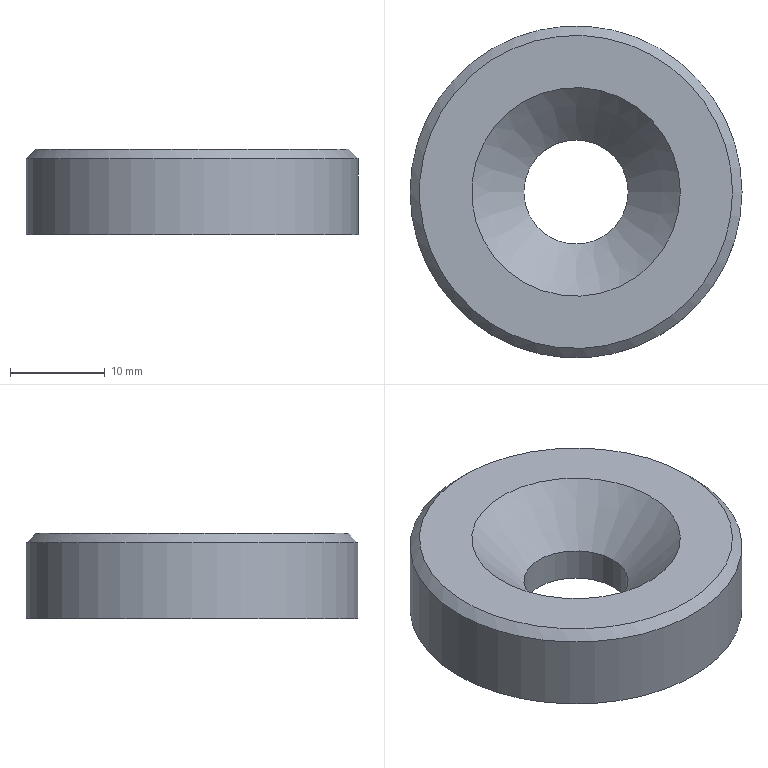Component | NX | END_CAP | 1 solid | 6 faces | box 35 x 35 x 9 mm | volume 7053 mm3 | plane 2 | cylinder 2 | cone 2 | commonest cylinder face diameters 35 x1 11 x1
STEP:
#1=CARTESIAN_POINT('',(0.,0.,0.));
#2=DIRECTION('',(0.,0.,1.));
#3=DIRECTION('',(1.,0.,0.));
#4=AXIS2_PLACEMENT_3D('',#1,#2,#3);
#5=CARTESIAN_POINT('',(16.5,0.,237.));
#6=VERTEX_POINT('',#5);
#7=CARTESIAN_POINT('',(-0.,0.,237.));
#8=DIRECTION('',(0.,0.,1.));
#9=DIRECTION('',(1.,0.,0.));
#10=AXIS2_PLACEMENT_3D('',#7,#8,#9);
#11=CIRCLE('',#10,16.5);
#12=CARTESIAN_POINT('',(-0.,0.,237.));
#13=DIRECTION('',(0.,0.,1.));
#14=DIRECTION('',(1.,0.,0.));
#15=AXIS2_PLACEMENT_3D('',#12,#13,#14);
#16=PLANE('',#15);
#17=CARTESIAN_POINT('',(0.,0.));
#18=DIRECTION('',(1.,0.));
#19=AXIS2_PLACEMENT_2D('',#17,#18);
#20=CIRCLE('',#19,16.5);
#21=(GEOMETRIC_REPRESENTATION_CONTEXT(2)PARAMETRIC_REPRESENTATION_CONTEXT()REPRESENTATION_CONTEXT('',''));
#22=DEFINITIONAL_REPRESENTATION('',(#20),#21);
#23=PCURVE('',#16,#22);
#24=CARTESIAN_POINT('',(-0.,0.,236.));
#25=DIRECTION('',(0.,0.,-1.));
#26=DIRECTION('',(-1.,0.,0.));
#27=AXIS2_PLACEMENT_3D('',#24,#25,#26);
#28=CONICAL_SURFACE('',#27,17.5,0.7854);
#29=CARTESIAN_POINT('',(9.425,-1.));
#30=DIRECTION('',(-1.,0.));
#31=VECTOR('',#30,1.);
#32=LINE('',#29,#31);
#33=(GEOMETRIC_REPRESENTATION_CONTEXT(2)PARAMETRIC_REPRESENTATION_CONTEXT()REPRESENTATION_CONTEXT('',''));
#34=DEFINITIONAL_REPRESENTATION('',(#32),#33);
#35=PCURVE('',#28,#34);
#36=SURFACE_CURVE('',#11,(#23,#35),.PCURVE_S1.);
#37=EDGE_CURVE('',#6,#6,#36,.T.);
#38=ORIENTED_EDGE('',*,*,#37,.T.);
#39=EDGE_LOOP('',(#38));
#40=FACE_BOUND('',#39,.T.);
#41=CARTESIAN_POINT('',(11.,0.,237.));
#42=VERTEX_POINT('',#41);
#43=CARTESIAN_POINT('',(-0.,0.,237.));
#44=DIRECTION('',(0.,0.,-1.));
#45=DIRECTION('',(1.,0.,0.));
#46=AXIS2_PLACEMENT_3D('',#43,#44,#45);
#47=CIRCLE('',#46,11.);
#48=CARTESIAN_POINT('',(11.,0.));
#49=CARTESIAN_POINT('',(11.,-19.053));
#50=CARTESIAN_POINT('',(-5.5,-9.526));
#51=CARTESIAN_POINT('',(-22.,-0.));
#52=CARTESIAN_POINT('',(-5.5,9.526));
#53=CARTESIAN_POINT('',(11.,19.053));
#54=CARTESIAN_POINT('',(11.,0.));
#55=(BOUNDED_CURVE()B_SPLINE_CURVE(2,(#48,#49,#50,#51,#52,#53,#54),.UNSPECIFIED.,.T.,.F.)B_SPLINE_CURVE_WITH_KNOTS((1,2,2,2,2,1),(-2.094,0.,2.094,4.189,6.283,8.378),.UNSPECIFIED.)CURVE()GEOMETRIC_REPRESENTATION_ITEM()RATIONAL_B_SPLINE_CURVE((1.,0.5,1.,0.5,1.,0.5,1.))REPRESENTATION_ITEM(''));
#56=(GEOMETRIC_REPRESENTATION_CONTEXT(2)PARAMETRIC_REPRESENTATION_CONTEXT()REPRESENTATION_CONTEXT('',''));
#57=DEFINITIONAL_REPRESENTATION('',(#55),#56);
#58=PCURVE('',#16,#57);
#59=CARTESIAN_POINT('',(-0.,0.,237.));
#60=DIRECTION('',(0.,0.,1.));
#61=DIRECTION('',(1.,0.,0.));
#62=AXIS2_PLACEMENT_3D('',#59,#60,#61);
#63=CONICAL_SURFACE('',#62,11.,0.7854);
#64=CARTESIAN_POINT('',(6.283,0.));
#65=DIRECTION('',(-1.,0.));
#66=VECTOR('',#65,1.);
#67=LINE('',#64,#66);
#68=(GEOMETRIC_REPRESENTATION_CONTEXT(2)PARAMETRIC_REPRESENTATION_CONTEXT()REPRESENTATION_CONTEXT('',''));
#69=DEFINITIONAL_REPRESENTATION('',(#67),#68);
#70=PCURVE('',#63,#69);
#71=SURFACE_CURVE('',#47,(#58,#70),.PCURVE_S1.);
#72=EDGE_CURVE('',#42,#42,#71,.T.);
#73=ORIENTED_EDGE('',*,*,#72,.T.);
#74=EDGE_LOOP('',(#73));
#75=FACE_BOUND('',#74,.T.);
#76=ADVANCED_FACE('',(#40,#75),#16,.T.);
#77=CARTESIAN_POINT('',(5.5,0.,228.));
#78=VERTEX_POINT('',#77);
#79=CARTESIAN_POINT('',(-0.,0.,228.));
#80=DIRECTION('',(0.,0.,1.));
#81=DIRECTION('',(1.,0.,0.));
#82=AXIS2_PLACEMENT_3D('',#79,#80,#81);
#83=CIRCLE('',#82,5.5);
#84=CARTESIAN_POINT('',(-0.,0.,228.));
#85=DIRECTION('',(0.,0.,-1.));
#86=DIRECTION('',(-1.,0.,0.));
#87=AXIS2_PLACEMENT_3D('',#84,#85,#86);
#88=PLANE('',#87);
#89=CARTESIAN_POINT('',(-5.5,0.));
#90=CARTESIAN_POINT('',(-5.5,9.526));
#91=CARTESIAN_POINT('',(2.75,4.763));
#92=CARTESIAN_POINT('',(11.,0.));
#93=CARTESIAN_POINT('',(2.75,-4.763));
#94=CARTESIAN_POINT('',(-5.5,-9.526));
#95=CARTESIAN_POINT('',(-5.5,0.));
#96=(BOUNDED_CURVE()B_SPLINE_CURVE(2,(#89,#90,#91,#92,#93,#94,#95),.UNSPECIFIED.,.T.,.F.)B_SPLINE_CURVE_WITH_KNOTS((1,2,2,2,2,1),(-2.094,0.,2.094,4.189,6.283,8.378),.UNSPECIFIED.)CURVE()GEOMETRIC_REPRESENTATION_ITEM()RATIONAL_B_SPLINE_CURVE((1.,0.5,1.,0.5,1.,0.5,1.))REPRESENTATION_ITEM(''));
#97=(GEOMETRIC_REPRESENTATION_CONTEXT(2)PARAMETRIC_REPRESENTATION_CONTEXT()REPRESENTATION_CONTEXT('',''));
#98=DEFINITIONAL_REPRESENTATION('',(#96),#97);
#99=PCURVE('',#88,#98);
#100=CARTESIAN_POINT('',(-0.,0.,228.));
#101=DIRECTION('',(0.,0.,1.));
#102=DIRECTION('',(1.,0.,0.));
#103=AXIS2_PLACEMENT_3D('',#100,#101,#102);
#104=CYLINDRICAL_SURFACE('',#103,5.5);
#105=CARTESIAN_POINT('',(0.,0.));
#106=DIRECTION('',(1.,0.));
#107=VECTOR('',#106,1.);
#108=LINE('',#105,#107);
#109=(GEOMETRIC_REPRESENTATION_CONTEXT(2)PARAMETRIC_REPRESENTATION_CONTEXT()REPRESENTATION_CONTEXT('',''));
#110=DEFINITIONAL_REPRESENTATION('',(#108),#109);
#111=PCURVE('',#104,#110);
#112=SURFACE_CURVE('',#83,(#99,#111),.PCURVE_S1.);
#113=EDGE_CURVE('',#78,#78,#112,.T.);
#114=ORIENTED_EDGE('',*,*,#113,.T.);
#115=EDGE_LOOP('',(#114));
#116=FACE_BOUND('',#115,.T.);
#117=CARTESIAN_POINT('',(17.5,0.,228.));
#118=VERTEX_POINT('',#117);
#119=CARTESIAN_POINT('',(-0.,0.,228.));
#120=DIRECTION('',(0.,0.,1.));
#121=DIRECTION('',(1.,0.,0.));
#122=AXIS2_PLACEMENT_3D('',#119,#120,#121);
#123=CIRCLE('',#122,17.5);
#124=CARTESIAN_POINT('',(-17.5,0.));
#125=CARTESIAN_POINT('',(-17.5,30.311));
#126=CARTESIAN_POINT('',(8.75,15.155));
#127=CARTESIAN_POINT('',(35.,0.));
#128=CARTESIAN_POINT('',(8.75,-15.155));
#129=CARTESIAN_POINT('',(-17.5,-30.311));
#130=CARTESIAN_POINT('',(-17.5,0.));
#131=(BOUNDED_CURVE()B_SPLINE_CURVE(2,(#124,#125,#126,#127,#128,#129,#130),.UNSPECIFIED.,.T.,.F.)B_SPLINE_CURVE_WITH_KNOTS((1,2,2,2,2,1),(-2.094,0.,2.094,4.189,6.283,8.378),.UNSPECIFIED.)CURVE()GEOMETRIC_REPRESENTATION_ITEM()RATIONAL_B_SPLINE_CURVE((1.,0.5,1.,0.5,1.,0.5,1.))REPRESENTATION_ITEM(''));
#132=(GEOMETRIC_REPRESENTATION_CONTEXT(2)PARAMETRIC_REPRESENTATION_CONTEXT()REPRESENTATION_CONTEXT('',''));
#133=DEFINITIONAL_REPRESENTATION('',(#131),#132);
#134=PCURVE('',#88,#133);
#135=CARTESIAN_POINT('',(-0.,0.,228.));
#136=DIRECTION('',(0.,0.,1.));
#137=DIRECTION('',(1.,0.,0.));
#138=AXIS2_PLACEMENT_3D('',#135,#136,#137);
#139=CYLINDRICAL_SURFACE('',#138,17.5);
#140=CARTESIAN_POINT('',(0.,0.));
#141=DIRECTION('',(1.,0.));
#142=VECTOR('',#141,1.);
#143=LINE('',#140,#142);
#144=(GEOMETRIC_REPRESENTATION_CONTEXT(2)PARAMETRIC_REPRESENTATION_CONTEXT()REPRESENTATION_CONTEXT('',''));
#145=DEFINITIONAL_REPRESENTATION('',(#143),#144);
#146=PCURVE('',#139,#145);
#147=SURFACE_CURVE('',#123,(#134,#146),.PCURVE_S1.);
#148=EDGE_CURVE('',#118,#118,#147,.T.);
#149=ORIENTED_EDGE('',*,*,#148,.F.);
#150=EDGE_LOOP('',(#149));
#151=FACE_BOUND('',#150,.T.);
#152=ADVANCED_FACE('',(#116,#151),#88,.T.);
#153=CARTESIAN_POINT('',(17.5,0.,236.));
#154=VERTEX_POINT('',#153);
#155=CARTESIAN_POINT('',(-0.,0.,236.));
#156=DIRECTION('',(0.,0.,-1.));
#157=DIRECTION('',(1.,0.,0.));
#158=AXIS2_PLACEMENT_3D('',#155,#156,#157);
#159=CIRCLE('',#158,17.5);
#160=CARTESIAN_POINT('',(6.283,8.));
#161=DIRECTION('',(-1.,0.));
#162=VECTOR('',#161,1.);
#163=LINE('',#160,#162);
#164=(GEOMETRIC_REPRESENTATION_CONTEXT(2)PARAMETRIC_REPRESENTATION_CONTEXT()REPRESENTATION_CONTEXT('',''));
#165=DEFINITIONAL_REPRESENTATION('',(#163),#164);
#166=PCURVE('',#139,#165);
#167=CARTESIAN_POINT('',(3.142,0.));
#168=DIRECTION('',(1.,0.));
#169=VECTOR('',#168,1.);
#170=LINE('',#167,#169);
#171=(GEOMETRIC_REPRESENTATION_CONTEXT(2)PARAMETRIC_REPRESENTATION_CONTEXT()REPRESENTATION_CONTEXT('',''));
#172=DEFINITIONAL_REPRESENTATION('',(#170),#171);
#173=PCURVE('',#28,#172);
#174=SURFACE_CURVE('',#159,(#166,#173),.PCURVE_S1.);
#175=EDGE_CURVE('',#154,#154,#174,.T.);
#176=ORIENTED_EDGE('',*,*,#175,.T.);
#177=CARTESIAN_POINT('',(17.5,0.,228.));
#178=CARTESIAN_POINT('',(17.5,0.,236.));
#179=B_SPLINE_CURVE_WITH_KNOTS('',1,(#177,#178),.UNSPECIFIED.,.F.,.F.,(2,2),(0.,8.),.PIECEWISE_BEZIER_KNOTS.);
#180=CARTESIAN_POINT('',(0.,0.));
#181=DIRECTION('',(0.,1.));
#182=VECTOR('',#181,1.);
#183=LINE('',#180,#182);
#184=(GEOMETRIC_REPRESENTATION_CONTEXT(2)PARAMETRIC_REPRESENTATION_CONTEXT()REPRESENTATION_CONTEXT('',''));
#185=DEFINITIONAL_REPRESENTATION('',(#183),#184);
#186=PCURVE('',#139,#185);
#187=CARTESIAN_POINT('',(6.283,0.));
#188=DIRECTION('',(0.,1.));
#189=VECTOR('',#188,1.);
#190=LINE('',#187,#189);
#191=(GEOMETRIC_REPRESENTATION_CONTEXT(2)PARAMETRIC_REPRESENTATION_CONTEXT()REPRESENTATION_CONTEXT('',''));
#192=DEFINITIONAL_REPRESENTATION('',(#190),#191);
#193=PCURVE('',#139,#192);
#194=SEAM_CURVE('',#179,(#186,#193),.PCURVE_S1.);
#195=EDGE_CURVE('',#118,#154,#194,.T.);
#196=ORIENTED_EDGE('',*,*,#195,.F.);
#197=ORIENTED_EDGE('',*,*,#148,.T.);
#198=ORIENTED_EDGE('',*,*,#195,.T.);
#199=EDGE_LOOP('',(#176,#196,#197,#198));
#200=FACE_BOUND('',#199,.T.);
#201=ADVANCED_FACE('',(#200),#139,.T.);
#202=CARTESIAN_POINT('',(5.5,0.,231.5));
#203=VERTEX_POINT('',#202);
#204=CARTESIAN_POINT('',(-0.,0.,231.5));
#205=DIRECTION('',(0.,0.,1.));
#206=DIRECTION('',(1.,0.,0.));
#207=AXIS2_PLACEMENT_3D('',#204,#205,#206);
#208=CIRCLE('',#207,5.5);
#209=CARTESIAN_POINT('',(0.,3.5));
#210=DIRECTION('',(1.,0.));
#211=VECTOR('',#210,1.);
#212=LINE('',#209,#211);
#213=(GEOMETRIC_REPRESENTATION_CONTEXT(2)PARAMETRIC_REPRESENTATION_CONTEXT()REPRESENTATION_CONTEXT('',''));
#214=DEFINITIONAL_REPRESENTATION('',(#212),#213);
#215=PCURVE('',#104,#214);
#216=CARTESIAN_POINT('',(0.,-5.5));
#217=DIRECTION('',(1.,0.));
#218=VECTOR('',#217,1.);
#219=LINE('',#216,#218);
#220=(GEOMETRIC_REPRESENTATION_CONTEXT(2)PARAMETRIC_REPRESENTATION_CONTEXT()REPRESENTATION_CONTEXT('',''));
#221=DEFINITIONAL_REPRESENTATION('',(#219),#220);
#222=PCURVE('',#63,#221);
#223=SURFACE_CURVE('',#208,(#215,#222),.PCURVE_S1.);
#224=EDGE_CURVE('',#203,#203,#223,.T.);
#225=ORIENTED_EDGE('',*,*,#224,.F.);
#226=CARTESIAN_POINT('',(5.5,0.,228.));
#227=CARTESIAN_POINT('',(5.5,0.,231.5));
#228=B_SPLINE_CURVE_WITH_KNOTS('',1,(#226,#227),.UNSPECIFIED.,.F.,.F.,(2,2),(0.,3.5),.PIECEWISE_BEZIER_KNOTS.);
#229=CARTESIAN_POINT('',(0.,0.));
#230=DIRECTION('',(0.,1.));
#231=VECTOR('',#230,1.);
#232=LINE('',#229,#231);
#233=(GEOMETRIC_REPRESENTATION_CONTEXT(2)PARAMETRIC_REPRESENTATION_CONTEXT()REPRESENTATION_CONTEXT('',''));
#234=DEFINITIONAL_REPRESENTATION('',(#232),#233);
#235=PCURVE('',#104,#234);
#236=CARTESIAN_POINT('',(6.283,0.));
#237=DIRECTION('',(0.,1.));
#238=VECTOR('',#237,1.);
#239=LINE('',#236,#238);
#240=(GEOMETRIC_REPRESENTATION_CONTEXT(2)PARAMETRIC_REPRESENTATION_CONTEXT()REPRESENTATION_CONTEXT('',''));
#241=DEFINITIONAL_REPRESENTATION('',(#239),#240);
#242=PCURVE('',#104,#241);
#243=SEAM_CURVE('',#228,(#235,#242),.PCURVE_S1.);
#244=EDGE_CURVE('',#78,#203,#243,.T.);
#245=ORIENTED_EDGE('',*,*,#244,.F.);
#246=ORIENTED_EDGE('',*,*,#113,.T.);
#247=ORIENTED_EDGE('',*,*,#244,.T.);
#248=EDGE_LOOP('',(#225,#245,#246,#247));
#249=FACE_BOUND('',#248,.F.);
#250=ADVANCED_FACE('',(#249),#104,.F.);
#251=ORIENTED_EDGE('',*,*,#224,.T.);
#252=CARTESIAN_POINT('',(5.5,0.,231.5));
#253=CARTESIAN_POINT('',(11.,0.,237.));
#254=B_SPLINE_CURVE_WITH_KNOTS('',1,(#252,#253),.UNSPECIFIED.,.F.,.F.,(2,2),(-7.778,0.),.PIECEWISE_BEZIER_KNOTS.);
#255=CARTESIAN_POINT('',(6.283,0.));
#256=DIRECTION('',(0.,1.));
#257=VECTOR('',#256,1.);
#258=LINE('',#255,#257);
#259=(GEOMETRIC_REPRESENTATION_CONTEXT(2)PARAMETRIC_REPRESENTATION_CONTEXT()REPRESENTATION_CONTEXT('',''));
#260=DEFINITIONAL_REPRESENTATION('',(#258),#259);
#261=PCURVE('',#63,#260);
#262=CARTESIAN_POINT('',(0.,0.));
#263=DIRECTION('',(0.,1.));
#264=VECTOR('',#263,1.);
#265=LINE('',#262,#264);
#266=(GEOMETRIC_REPRESENTATION_CONTEXT(2)PARAMETRIC_REPRESENTATION_CONTEXT()REPRESENTATION_CONTEXT('',''));
#267=DEFINITIONAL_REPRESENTATION('',(#265),#266);
#268=PCURVE('',#63,#267);
#269=SEAM_CURVE('',#254,(#261,#268),.PCURVE_S1.);
#270=EDGE_CURVE('',#203,#42,#269,.T.);
#271=ORIENTED_EDGE('',*,*,#270,.T.);
#272=ORIENTED_EDGE('',*,*,#72,.T.);
#273=ORIENTED_EDGE('',*,*,#270,.F.);
#274=EDGE_LOOP('',(#251,#271,#272,#273));
#275=FACE_BOUND('',#274,.F.);
#276=ADVANCED_FACE('',(#275),#63,.F.);
#277=ORIENTED_EDGE('',*,*,#37,.F.);
#278=CARTESIAN_POINT('',(16.5,0.,237.));
#279=CARTESIAN_POINT('',(17.5,0.,236.));
#280=B_SPLINE_CURVE_WITH_KNOTS('',1,(#278,#279),.UNSPECIFIED.,.F.,.F.,(2,2),(-1.414,0.),.PIECEWISE_BEZIER_KNOTS.);
#281=CARTESIAN_POINT('',(9.425,0.));
#282=DIRECTION('',(0.,1.));
#283=VECTOR('',#282,1.);
#284=LINE('',#281,#283);
#285=(GEOMETRIC_REPRESENTATION_CONTEXT(2)PARAMETRIC_REPRESENTATION_CONTEXT()REPRESENTATION_CONTEXT('',''));
#286=DEFINITIONAL_REPRESENTATION('',(#284),#285);
#287=PCURVE('',#28,#286);
#288=CARTESIAN_POINT('',(3.142,0.));
#289=DIRECTION('',(0.,1.));
#290=VECTOR('',#289,1.);
#291=LINE('',#288,#290);
#292=(GEOMETRIC_REPRESENTATION_CONTEXT(2)PARAMETRIC_REPRESENTATION_CONTEXT()REPRESENTATION_CONTEXT('',''));
#293=DEFINITIONAL_REPRESENTATION('',(#291),#292);
#294=PCURVE('',#28,#293);
#295=SEAM_CURVE('',#280,(#287,#294),.PCURVE_S1.);
#296=EDGE_CURVE('',#6,#154,#295,.T.);
#297=ORIENTED_EDGE('',*,*,#296,.T.);
#298=ORIENTED_EDGE('',*,*,#175,.F.);
#299=ORIENTED_EDGE('',*,*,#296,.F.);
#300=EDGE_LOOP('',(#277,#297,#298,#299));
#301=FACE_BOUND('',#300,.T.);
#302=ADVANCED_FACE('',(#301),#28,.T.);
#303=CLOSED_SHELL('',(#76,#152,#201,#250,#276,#302));
#304=MANIFOLD_SOLID_BREP('',#303);
#305=(LENGTH_UNIT()NAMED_UNIT(*)SI_UNIT(.MILLI.,.METRE.));
#306=UNCERTAINTY_MEASURE_WITH_UNIT(LENGTH_MEASURE(0.00001),#305,'','');
#307=(NAMED_UNIT(*)PLANE_ANGLE_UNIT()SI_UNIT($,.RADIAN.));
#308=(NAMED_UNIT(*)SI_UNIT($,.STERADIAN.)SOLID_ANGLE_UNIT());
#309=(GEOMETRIC_REPRESENTATION_CONTEXT(3)GLOBAL_UNCERTAINTY_ASSIGNED_CONTEXT((#306))GLOBAL_UNIT_ASSIGNED_CONTEXT((#305,#307,#308))REPRESENTATION_CONTEXT('',''));
#310=ADVANCED_BREP_SHAPE_REPRESENTATION('',(#4,#304),#309);